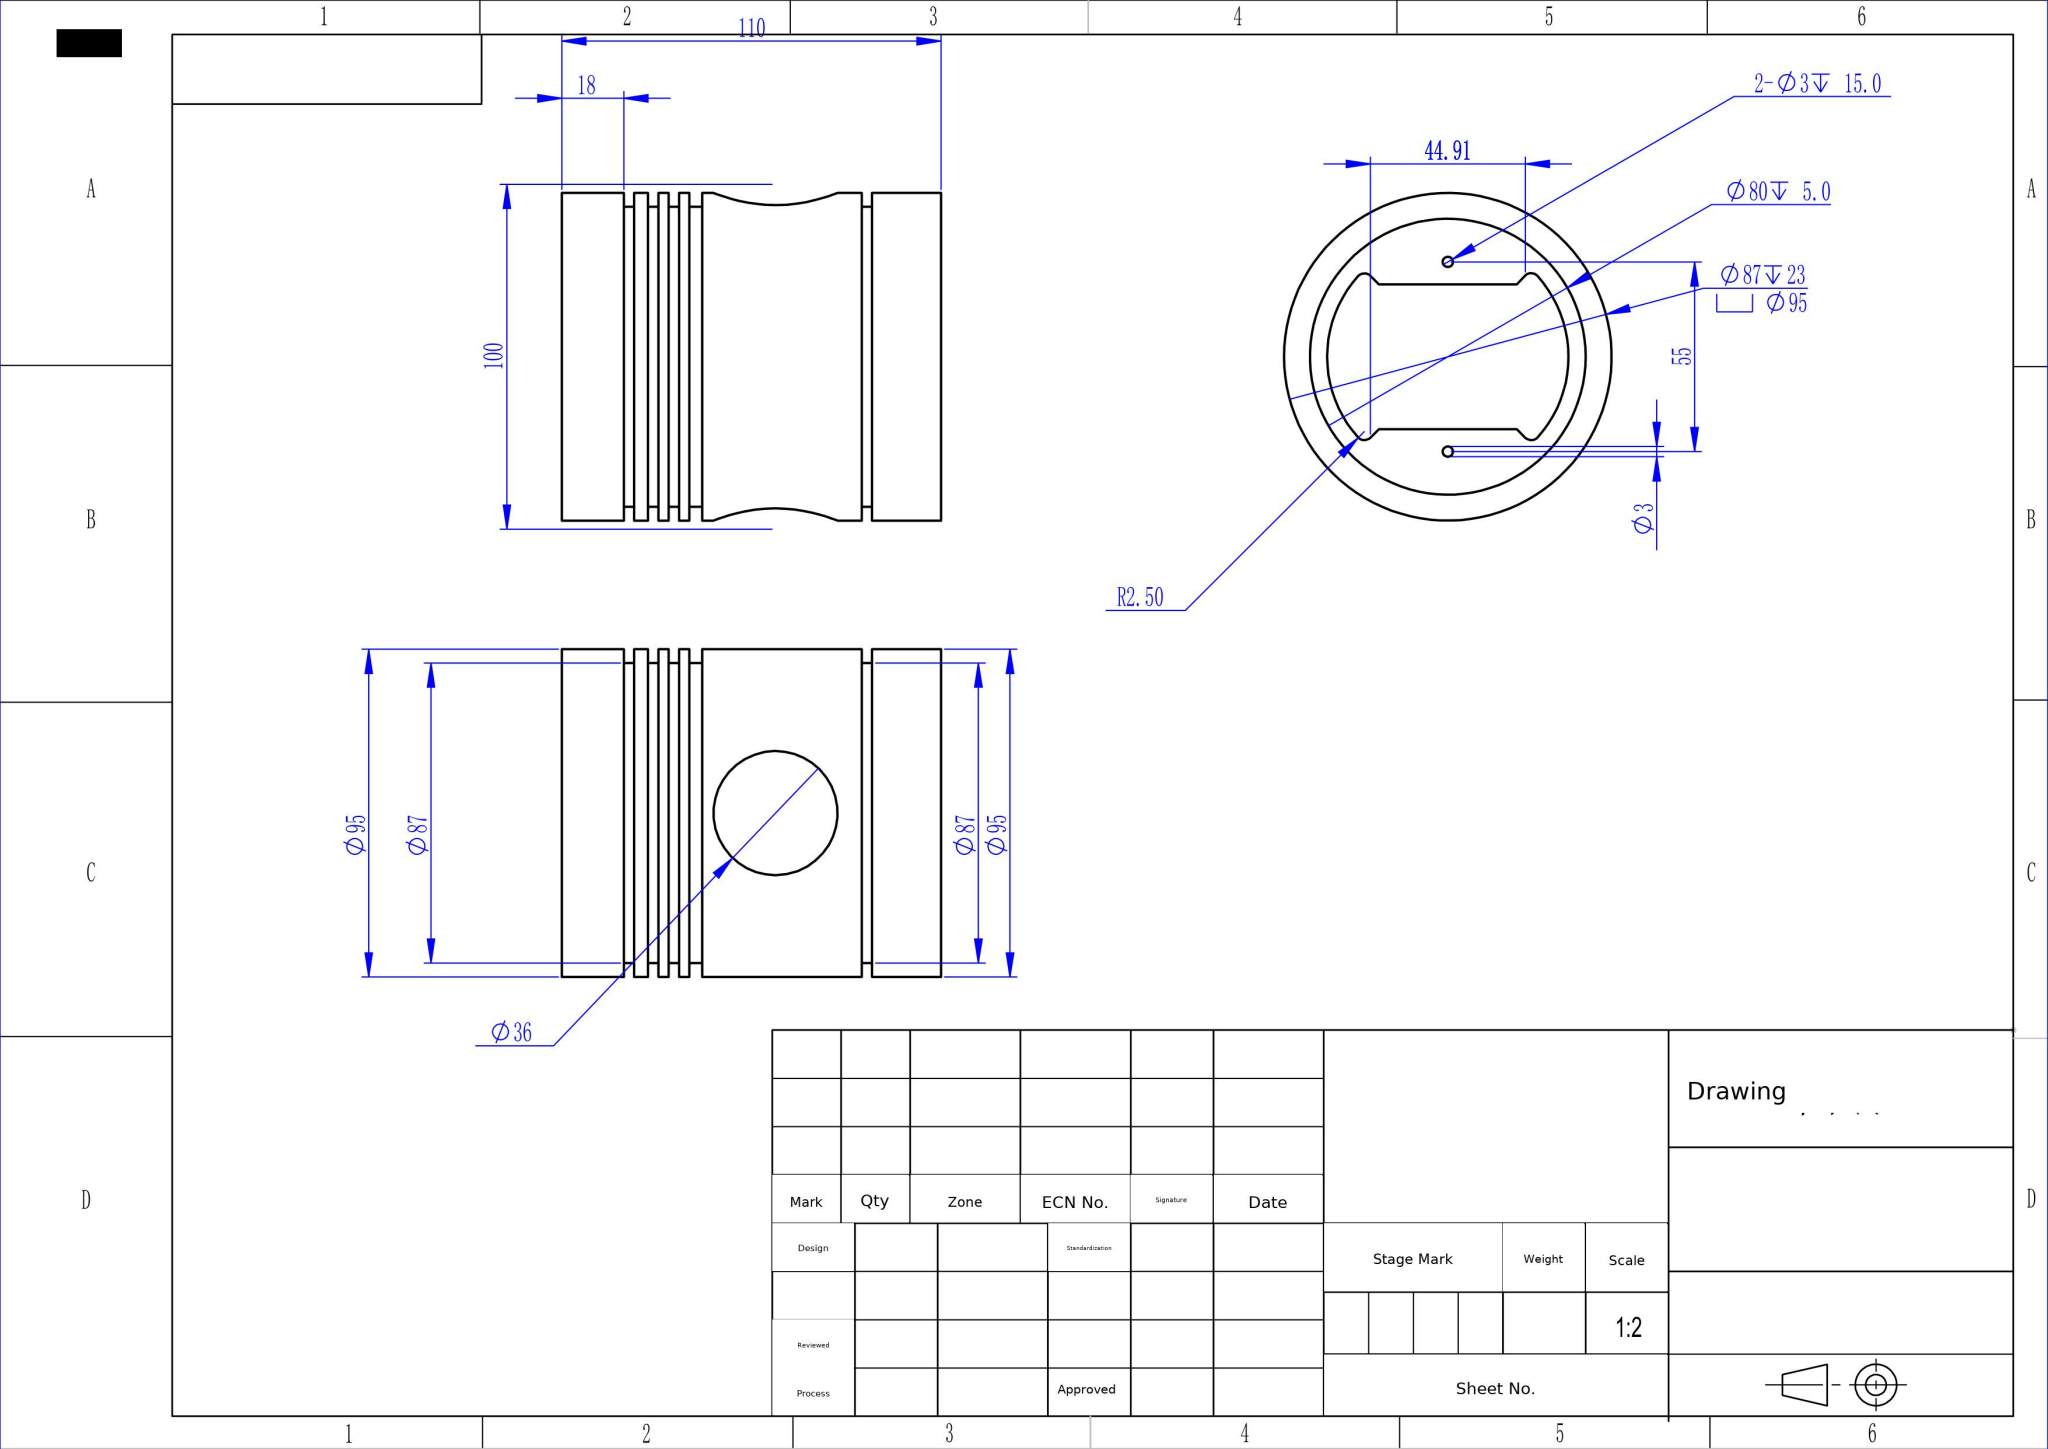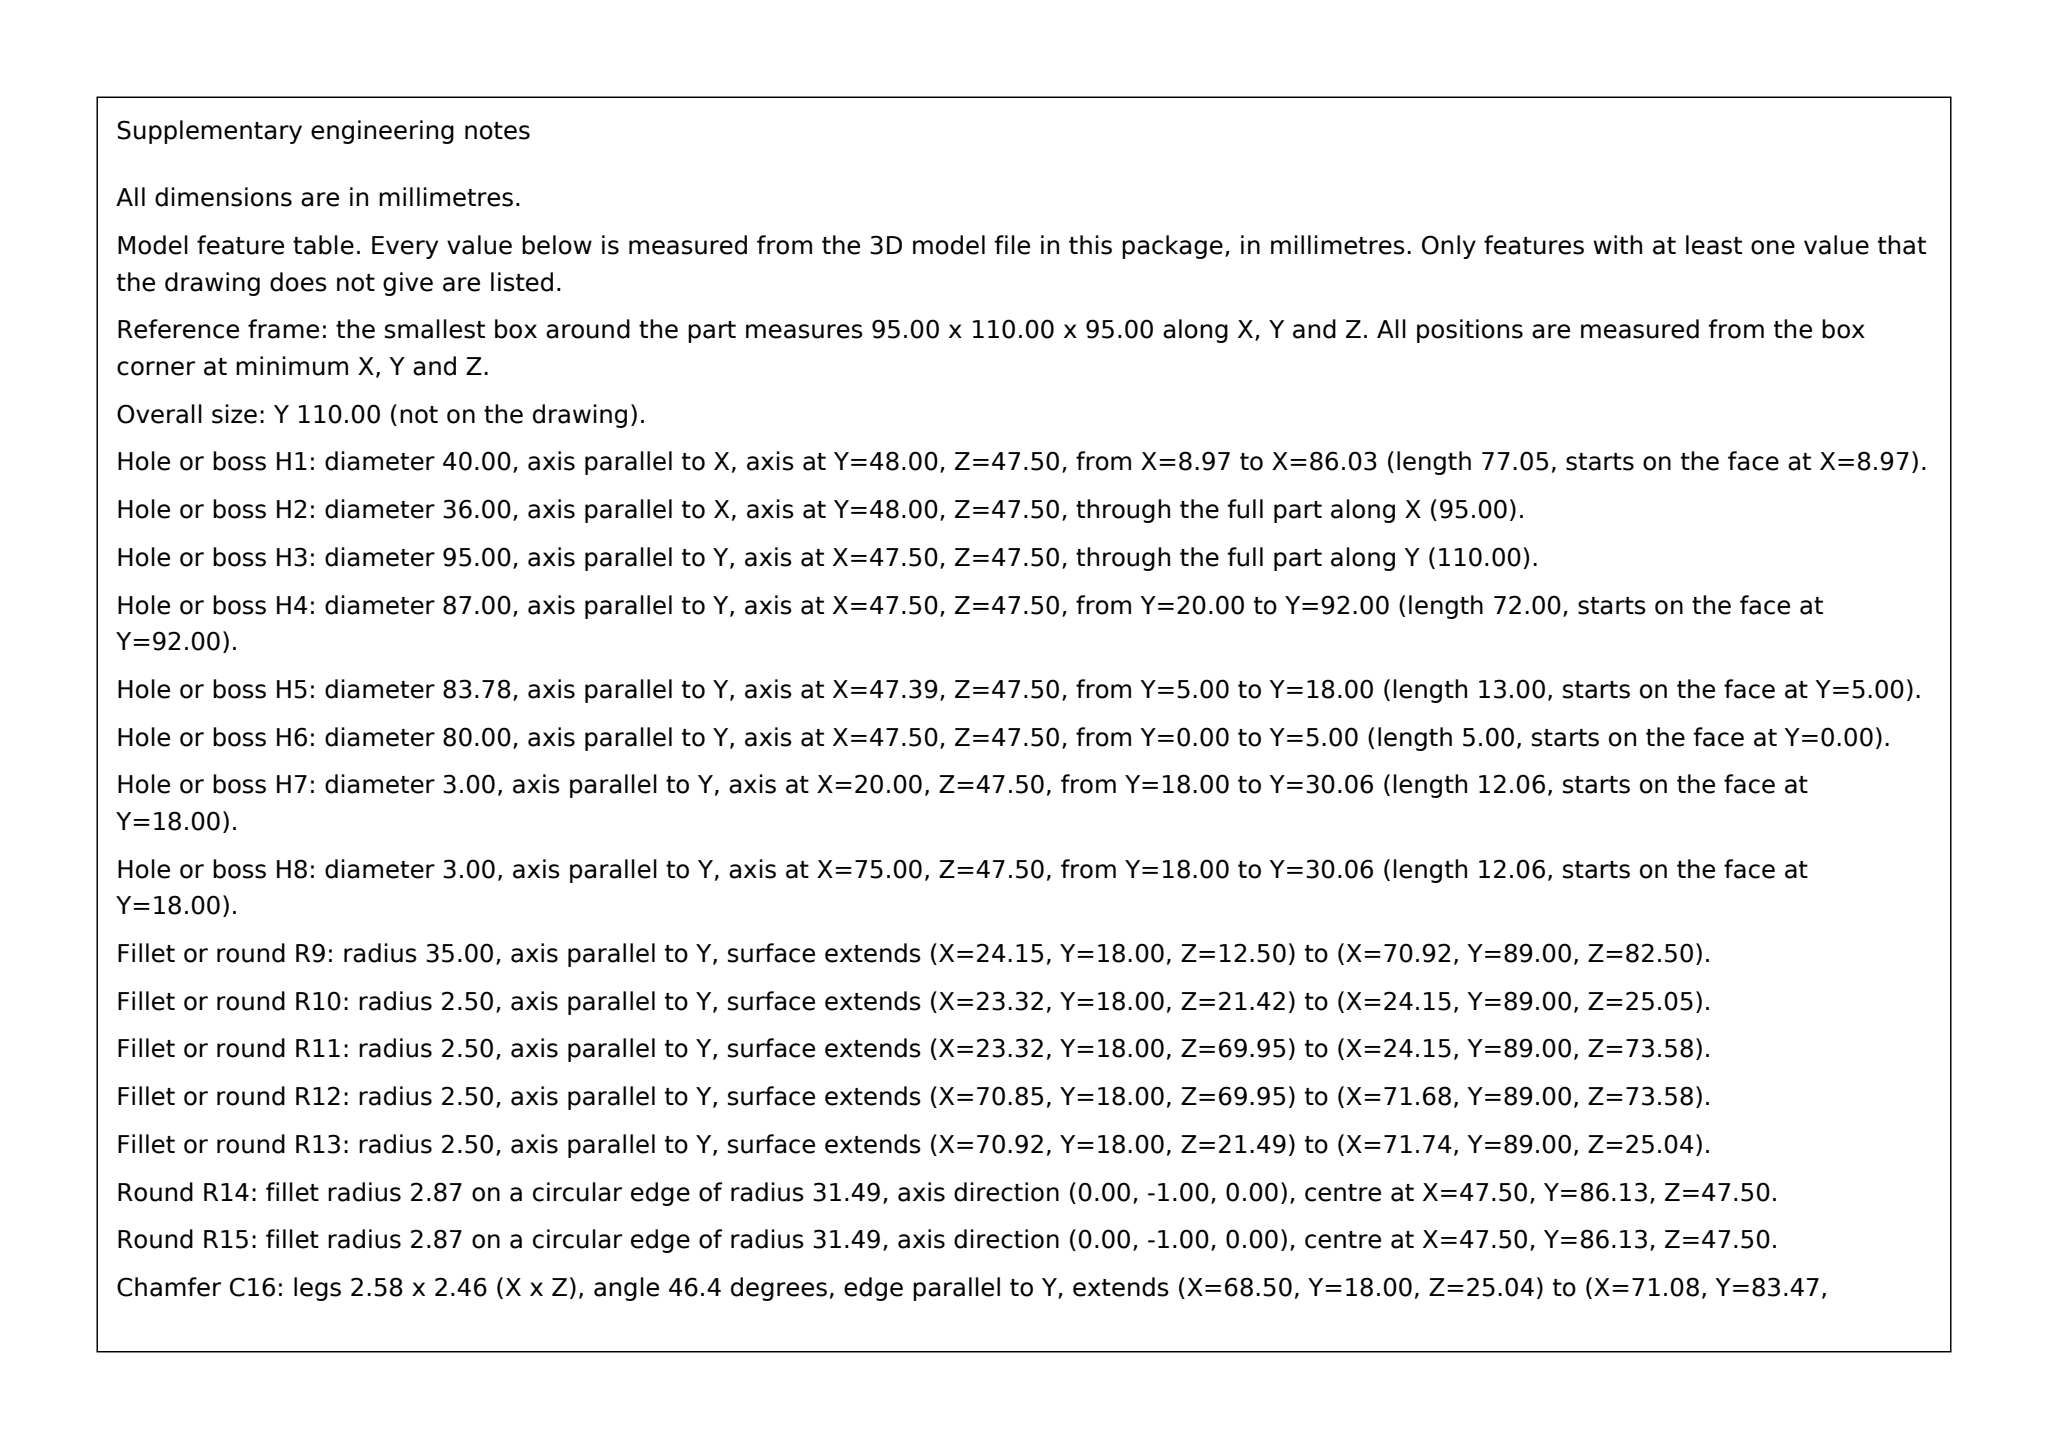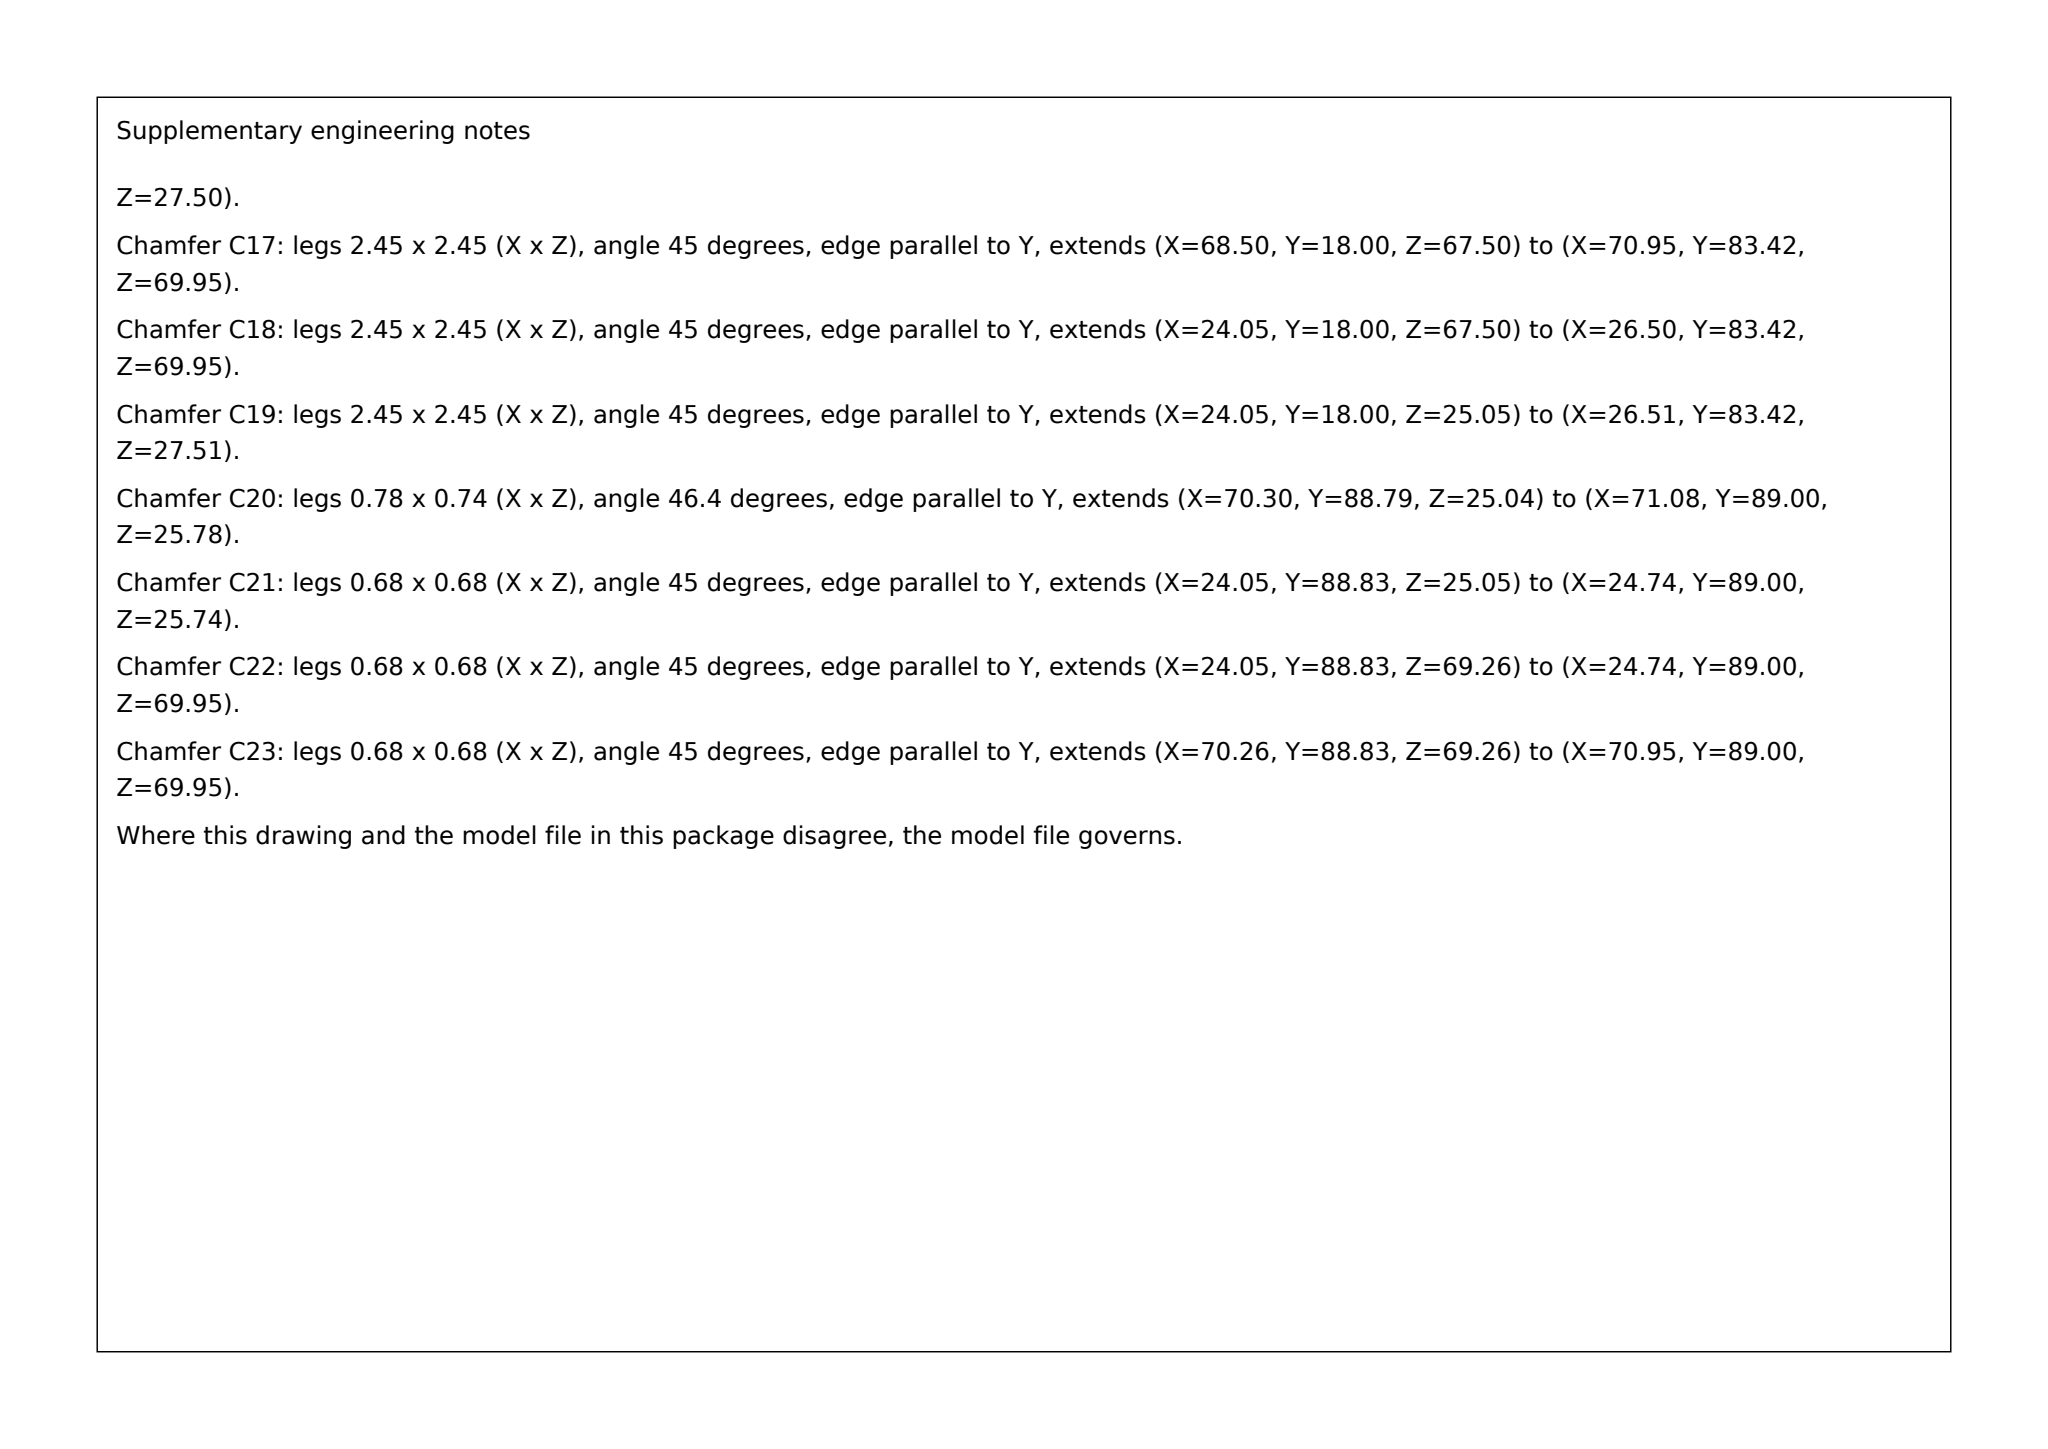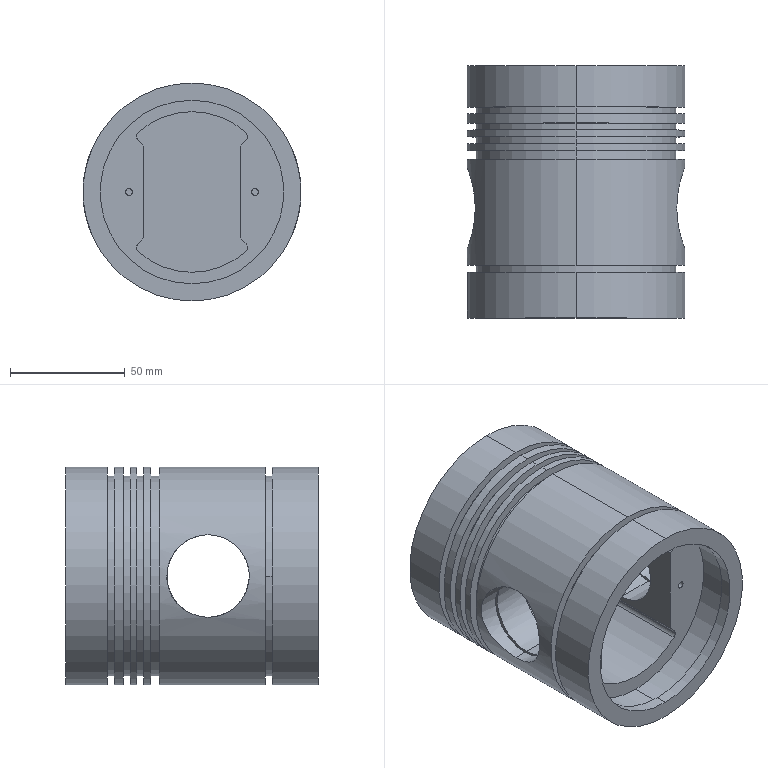Part | SolidWorks | mm | 1 solid | 85 faces | box 95 x 110 x 95 mm | volume 405541 mm3 | cylinder 52 | plane 29 | cone 2 | torus 2 | commonest cylinder face diameters 95 x12 87 x10 36 x8 5 x8 40 x4 3 x4 80 x2 83.784 x2
build123d program:
from build123d import *

# Parameters (mm, degrees)
SKETCH1_R           = 47.5
BOSS_EXTRUDE1_DEPTH = 110
SKETCH3_R           = 40
CUT_EXTRUDE1_DEPTH  = 5
SKETCH4_W           = 41.892
SKETCH4_H           = 13
CUT_EXTRUDE2_DEPTH  = 60
SKETCH9_W           = 4
SKETCH9_H           = 3
SKETCH9_H_2         = 3.762
SKETCH10_R          = 18
CUT_EXTRUDE3_DEPTH  = 50
SKETCH15_R          = 1.5
CUT_EXTRUDE4_DEPTH  = 15
SKETCH16_W          = 1
SKETCH16_H          = 2
SKETCH17_W          = 4
SKETCH17_H          = 3
SKETCH18_R          = 20
CUT_EXTRUDE5_DEPTH  = 11


with BuildPart() as part:
    # Sketch1 → Boss-Extrude1 (new body)
    with BuildSketch(Plane(origin=(0, 0, 0), x_dir=(1, 0, 0), z_dir=(0, 1, 0))):
        with Locations(Location((0, 0, 0), (0, 0, 270))):
            Circle(SKETCH1_R)
    extrude(amount=BOSS_EXTRUDE1_DEPTH)

    # Sketch3 → Cut-Extrude1 (cut)
    with BuildSketch(Plane.XZ):
        with Locations(Location((0, 0, 0), (0, 0, 270))):
            Circle(SKETCH3_R)
    extrude(amount=-CUT_EXTRUDE1_DEPTH, mode=Mode.SUBTRACT)

    # Sketch4 → Cut-Revolve4 (revolve, cut)
    with BuildSketch(Plane.XY, mode=Mode.PRIVATE) as cut_revolve4_sk:
        with Locations((-21.054, 11.5)):
            Rectangle(SKETCH4_W, SKETCH4_H)
    revolve(cut_revolve4_sk.sketch.rotate(Axis((-0.108, 18, 0), (0, -1, 0)), 270), axis=Axis((-0.108, 18, 0), (0, -1, 0)), mode=Mode.SUBTRACT)

    # Sketch6 → Cut-Extrude2 (cut)
    with BuildSketch(Plane.XZ.offset(-18)):
        with BuildLine():
            Line((21, 20), (21, -20))
            Line((21, -20), (23.584, -22.461))
            ThreePointArc((23.584, -22.461), (24.242, -24.272), (23.417, -26.012))
            ThreePointArc((23.417, -26.012), (0.04809, -35), (-23.346, -26.076))
            ThreePointArc((-23.346, -26.076), (-24.177, -24.283), (-23.446, -22.446))
            Line((-23.446, -22.446), (-20.994, -19.994))
            Line((-20.994, -19.994), (-21, 20))
            Line((-21, 20), (-23.446, 22.446))
            ThreePointArc((-23.446, 22.446), (-24.177, 24.283), (-23.346, 26.076))
            ThreePointArc((-23.346, 26.076), (0, 35), (23.346, 26.076))
            ThreePointArc((23.346, 26.076), (24.177, 24.283), (23.446, 22.446))
            Line((23.446, 22.446), (21, 20))
        make_face()
    extrude(amount=-CUT_EXTRUDE2_DEPTH, mode=Mode.SUBTRACT)

    # Sketch8 → Cut-Revolve5 (revolve, cut)
    with BuildSketch(Plane(origin=(0, 0, 0), x_dir=(0, 0, -1), z_dir=(1, 0, 0)), mode=Mode.PRIVATE) as cut_revolve5_sk:
        with BuildLine():
            Line((0, 78), (-20, 78))
            Line((-20, 78), (-32.635, 83.5))
            ThreePointArc((-32.635, 83.5), (-34.299, 86.716), (-31.49, 89))
            Line((-31.49, 89), (0, 89))
            Line((0, 89), (0, 78))
        make_face()
    revolve(cut_revolve5_sk.sketch.rotate(Axis((0, 69.757, 0), (0, 1, 0)), 180), axis=Axis((0, 69.757, 0), (0, 1, 0)), mode=Mode.SUBTRACT)

    # Sketch9 → Cut-Revolve6 (revolve, cut)
    with BuildSketch(Plane.XY, mode=Mode.PRIVATE) as cut_revolve6_sk:
        with Locations((-45.5, 90.5)):
            Rectangle(SKETCH9_W, SKETCH9_H)
        with Locations((-45.5, 83.5)):
            Rectangle(SKETCH9_W, SKETCH9_H)
        with Locations((-45.5, 77.5)):
            Rectangle(SKETCH9_W, SKETCH9_H)
        with Locations((-45.5, 71.119)):
            Rectangle(SKETCH9_W, SKETCH9_H_2)
    revolve(cut_revolve6_sk.sketch.rotate(Axis((0, 0, 0), (0, 1, 0)), 270), axis=Axis((0, 0, 0), (0, 1, 0)), mode=Mode.SUBTRACT)

    # Sketch10 → Cut-Extrude3 (cut, symmetric)
    with BuildSketch(Plane(origin=(0, 0, 0), x_dir=(0, 0, -1), z_dir=(1, 0, 0))):
        with Locations((0, 48)):
            Circle(SKETCH10_R)
    extrude(amount=CUT_EXTRUDE3_DEPTH, both=True, mode=Mode.SUBTRACT)

    # Sketch15 → Cut-Extrude4 (cut)
    with BuildSketch(Plane.XZ.offset(-18)):
        with Locations(Location((-27.5, 0, 0), (0, 0, 270))):
            Circle(SKETCH15_R)
        with Locations(Location((27.5, 0, 0), (0, 0, 270))):
            Circle(SKETCH15_R)
    extrude(amount=-CUT_EXTRUDE4_DEPTH, mode=Mode.SUBTRACT)

    # Sketch16 → Cut-Revolve8 (revolve, cut)
    with BuildSketch(Plane.XY):
        with Locations((38.026, 29)):
            Rectangle(SKETCH16_W, SKETCH16_H)
    cut_revolve8 = revolve(axis=Axis((21.5, 48, 0), (1, 0, 0)), mode=Mode.SUBTRACT)

    # Mirror1: Cut-Revolve8 across plane
    add(cut_revolve8.mirror(Plane(origin=(0, 0, 0), x_dir=(0, 0, 1), z_dir=(1, 0, 0))), mode=Mode.SUBTRACT)

    # Sketch17 → Cut-Revolve9 (revolve, cut)
    with BuildSketch(Plane.XY, mode=Mode.PRIVATE) as cut_revolve9_sk:
        with Locations((-45.5, 21.5)):
            Rectangle(SKETCH17_W, SKETCH17_H)
    revolve(cut_revolve9_sk.sketch.rotate(Axis((0, 58.899, 0), (0, -1, 0)), 90), axis=Axis((0, 58.899, 0), (0, -1, 0)), mode=Mode.SUBTRACT)

    # Sketch18 → Cut-Extrude5 (cut)
    with BuildSketch(Plane.XZ.offset(-78)):
        with BuildLine():
            Line((23.584, -22.461), (21, -20))
            Line((21, -20), (21, 20))
            Line((21, 20), (23.446, 22.446))
            ThreePointArc((23.446, 22.446), (24.177, 24.283), (23.346, 26.076))
            ThreePointArc((23.346, 26.076), (0, 35), (-23.346, 26.076))
            ThreePointArc((-23.346, 26.076), (-24.177, 24.283), (-23.446, 22.446))
            Line((-23.446, 22.446), (-21, 20))
            Line((-21, 20), (-20.994, -19.994))
            Line((-20.994, -19.994), (-23.446, -22.446))
            ThreePointArc((-23.446, -22.446), (-24.177, -24.283), (-23.346, -26.076))
            ThreePointArc((-23.346, -26.076), (0.04809, -35), (23.417, -26.012))
            ThreePointArc((23.417, -26.012), (24.242, -24.272), (23.584, -22.461))
        make_face()
        Circle(SKETCH18_R, mode=Mode.SUBTRACT)
    extrude(amount=-CUT_EXTRUDE5_DEPTH, mode=Mode.SUBTRACT)


solid = part.part